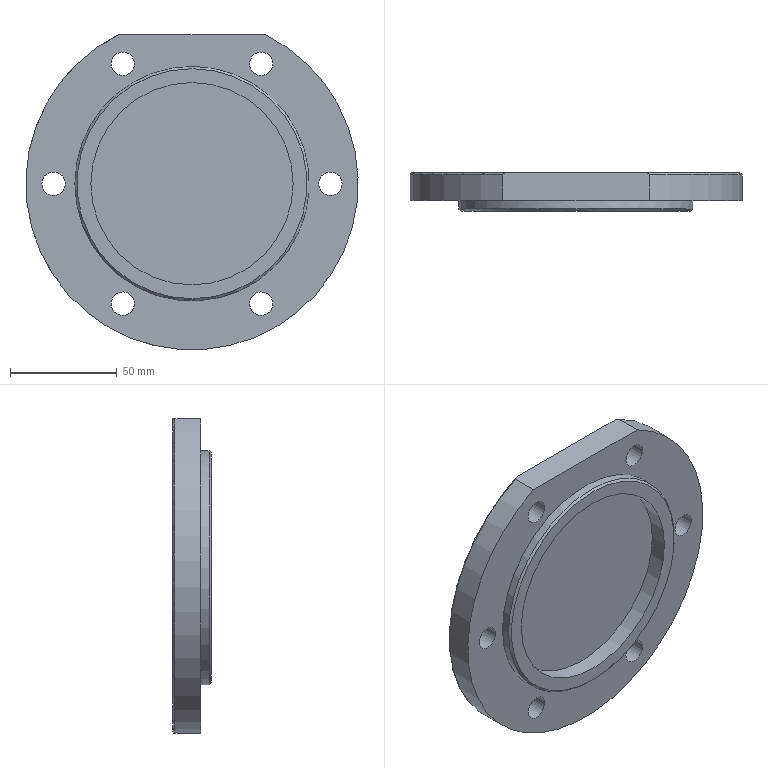Component | NX | END_CAP3 | 1 solid | 18 faces | volume 211081 mm3 | cylinder 10 | plane 6 | torus 1 | cone 1 | commonest cylinder face diameters 11 x6 156 x1 110 x1 95 x1 100 x1